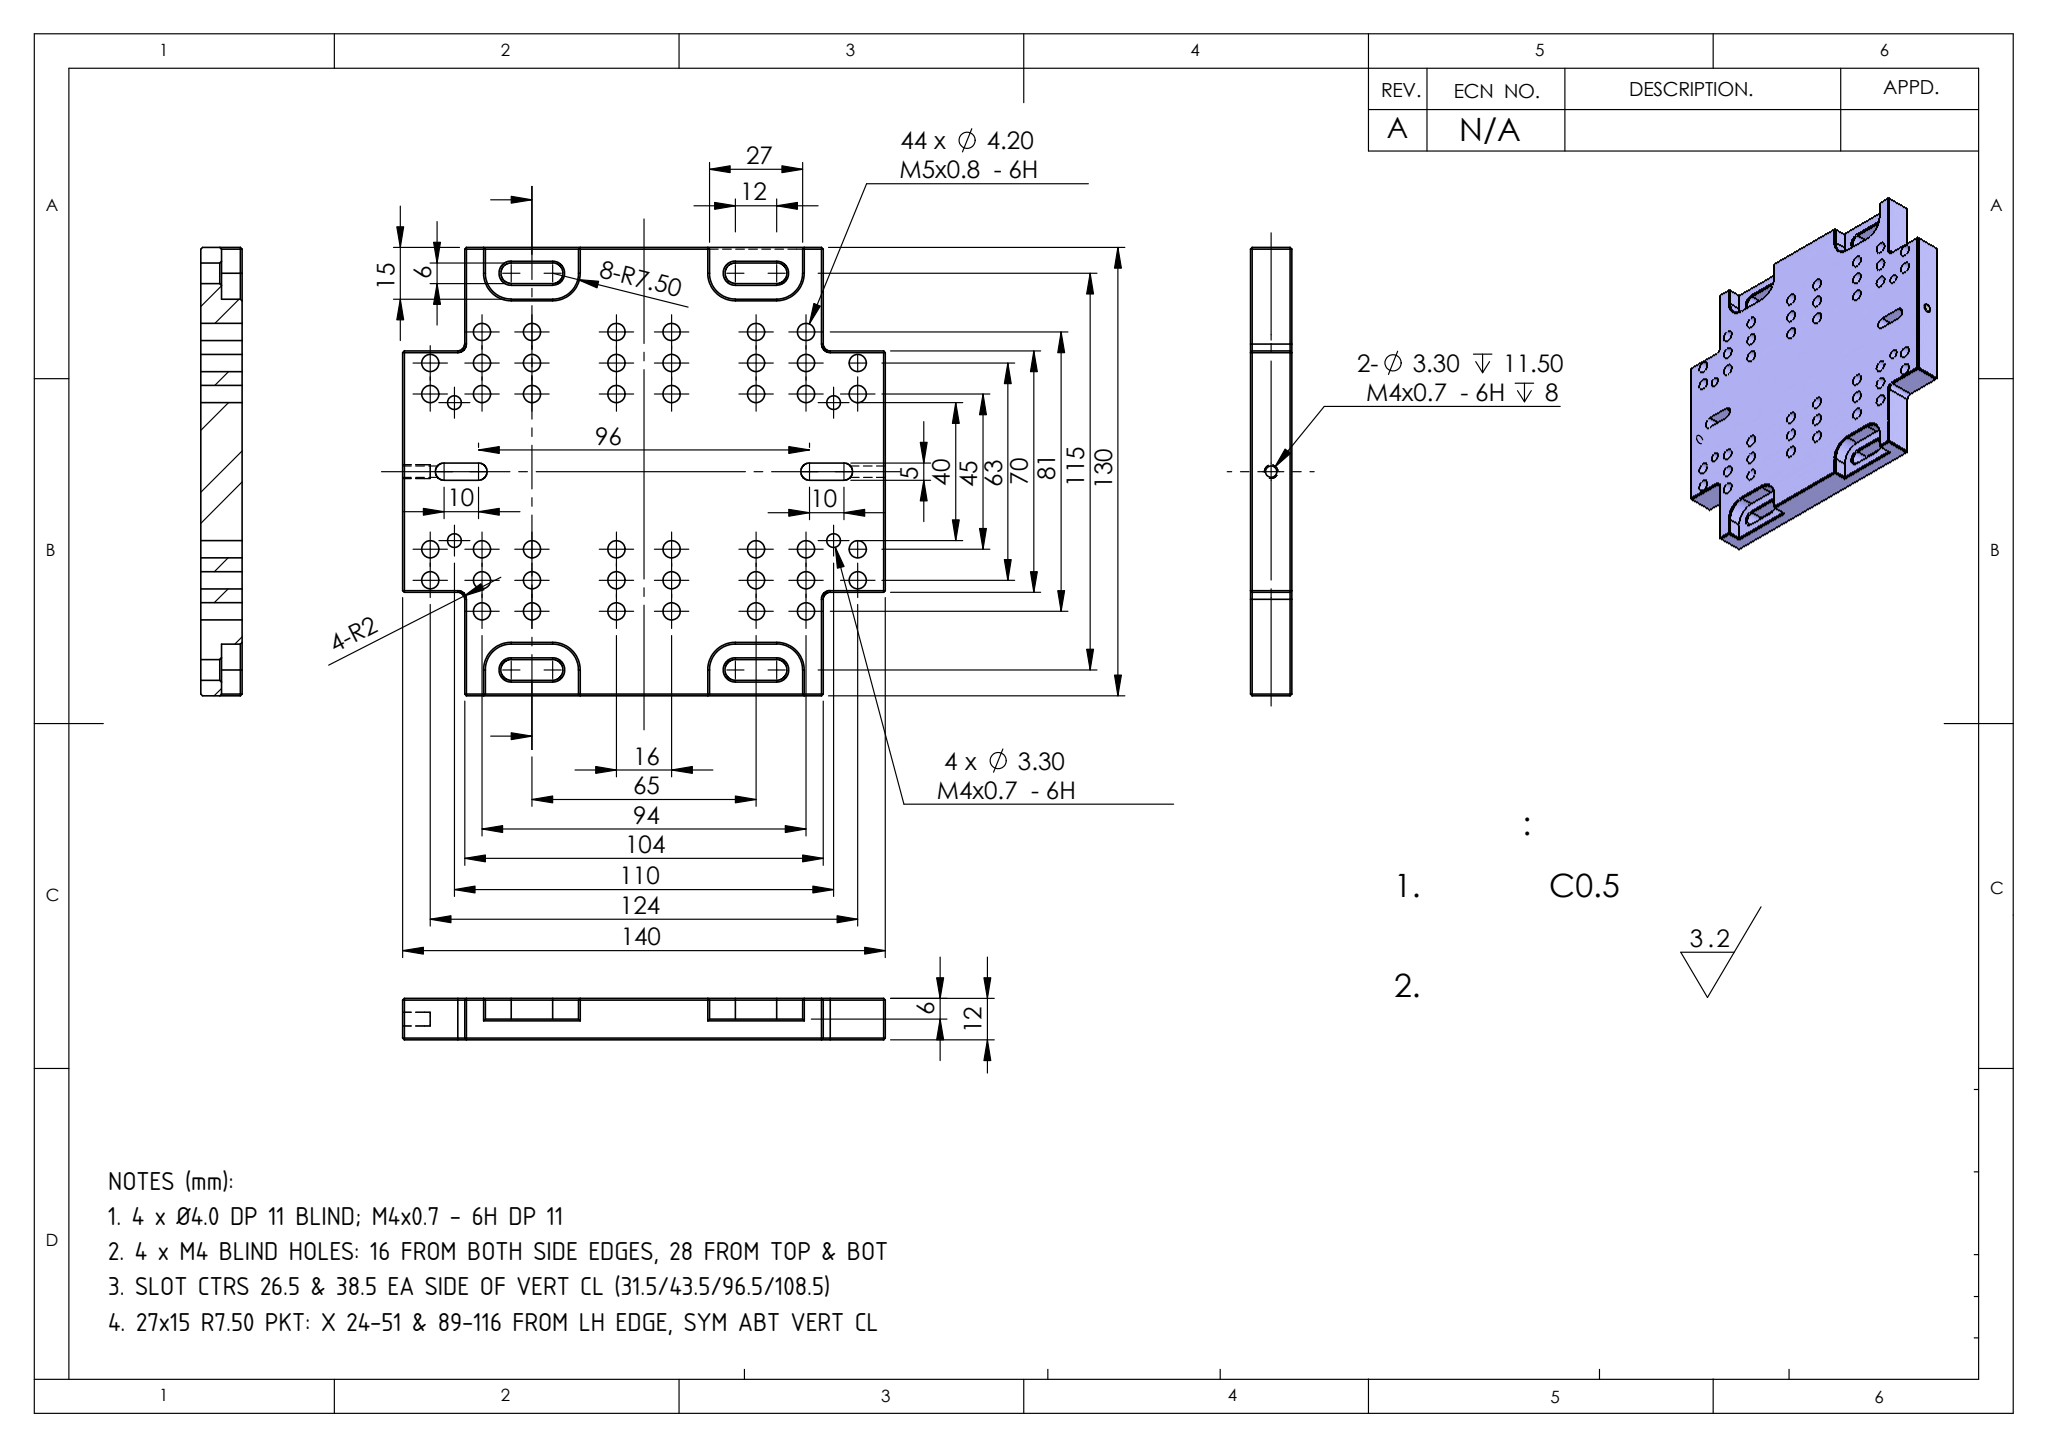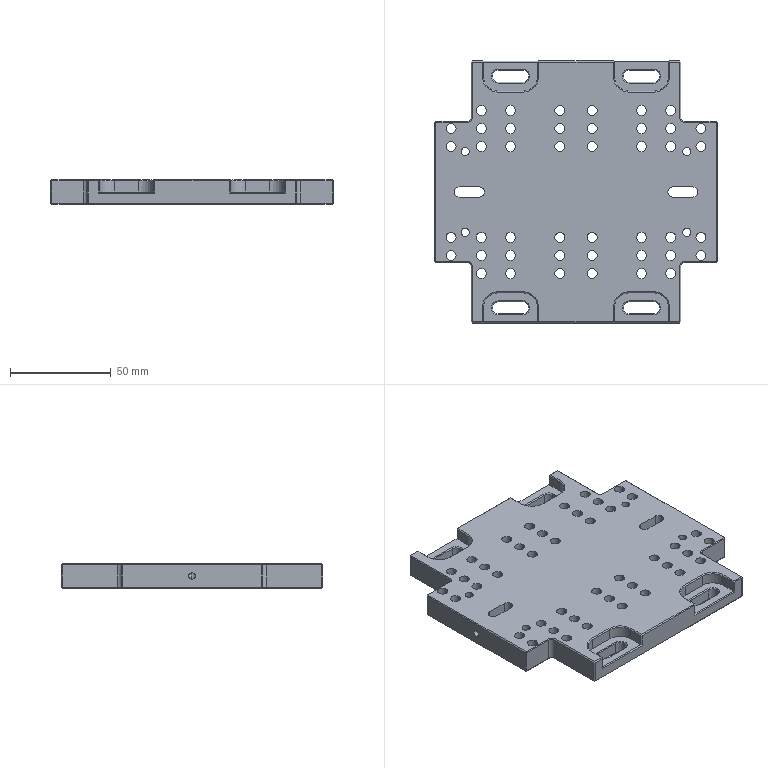Part | SolidWorks | mm | 1 solid | 291 faces | box 140 x 130 x 12 mm | volume 167973 mm3 | plane 133 | cylinder 130 | cone 28 | commonest cylinder face diameters 5 x94 4 x12 6 x12 15 x8 3.3 x4
Drawing notes:
4 x Ø4.0 DP 11 BLIND; M4x0.7 - 6H DP 11 | from the solid: cylinders dia 4.0, axis z, at (16,28),(16,102),(124,28),(124,102), length 11.0 in 12 thk plate
4 x M4 BLIND HOLES: 16 FROM BOTH SIDE EDGES, 28 FROM TOP & BOT | from the solid: x=16 & 124 (140-124=16); y=28 & 102 (130-102=28); bbox 140x130x12
SLOT CTRS 26.5 & 38.5 EA SIDE OF VERT CL (31.5/43.5/96.5/108.5) | from the solid: Ø6 slot-end cyls at x=31.5, 43.5, 96.5, 108.5; bbox x=140 so CL x=70
27x15 R7.50 PKT: X 24-51 & 89-116 FROM LH EDGE, SYM ABT VERT CL | from the solid: x-planes at 24, 51, 89, 116 bounding pockets; Ø15 c'bore ctrs 31.5/43.5/96.5/108.5